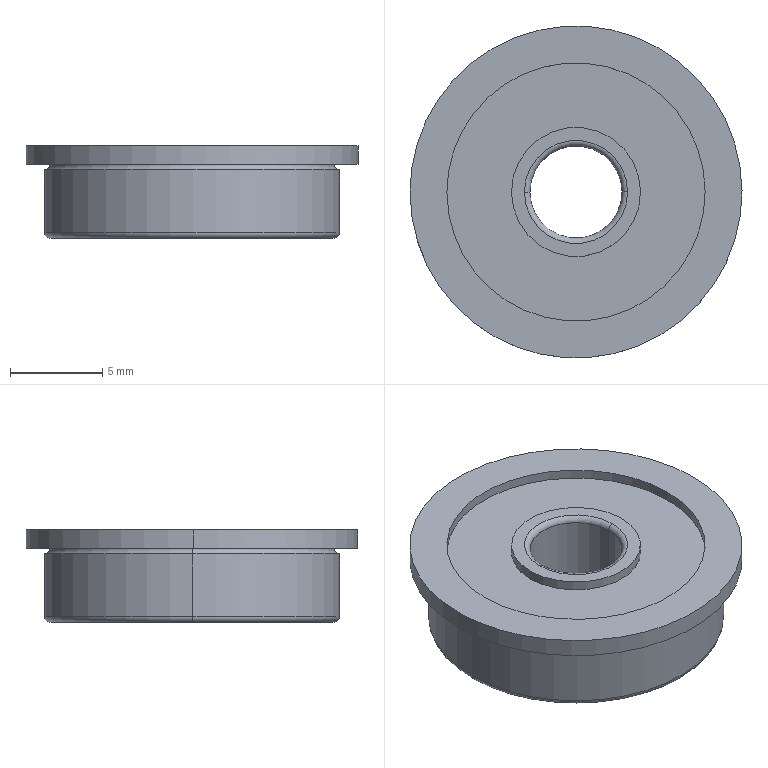Component | SolidWorks | SL010-LeftStreamline-1-1_SL010-PulleyAssembly-1-2_SL010-FL625ZZ-1-2 | 1 solid | 31 faces | box 18 x 18 x 5 mm | volume 827 mm3 | cylinder 14 | torus 10 | plane 7 | commonest cylinder face diameters 7 x4 14 x4 16 x2 18 x2 5 x2
STEP:
#1=COLOUR_RGB('',0.7922,0.8196,0.9333);
#2=FILL_AREA_STYLE_COLOUR('',#1);
#3=FILL_AREA_STYLE('',(#2));
#4=SURFACE_STYLE_FILL_AREA(#3);
#5=SURFACE_SIDE_STYLE('',(#4));
#6=SURFACE_STYLE_USAGE(.BOTH.,#5);
#7=PRESENTATION_STYLE_ASSIGNMENT((#6));
#8=CARTESIAN_POINT('',(-29.594,-5.329,-24.923));
#9=VERTEX_POINT('',#8);
#10=CARTESIAN_POINT('',(-29.618,-5.329,-24.923));
#11=VERTEX_POINT('',#10);
#12=CARTESIAN_POINT('',(-29.594,-5.329,-24.923));
#13=CARTESIAN_POINT('',(-29.594,-5.329,-24.92));
#14=CARTESIAN_POINT('',(-29.596,-5.329,-24.916));
#15=CARTESIAN_POINT('',(-29.6,-5.329,-24.912));
#16=CARTESIAN_POINT('',(-29.603,-5.329,-24.911));
#17=CARTESIAN_POINT('',(-29.609,-5.329,-24.911));
#18=CARTESIAN_POINT('',(-29.612,-5.329,-24.912));
#19=CARTESIAN_POINT('',(-29.617,-5.329,-24.916));
#20=CARTESIAN_POINT('',(-29.618,-5.329,-24.92));
#21=CARTESIAN_POINT('',(-29.618,-5.329,-24.923));
#22=B_SPLINE_CURVE_WITH_KNOTS('',3,(#12,#13,#14,#15,#16,#17,#18,#19,#20,#21),.UNSPECIFIED.,.F.,.F.,(4,2,2,2,4),(0.,0.7854,1.571,2.356,3.142),.UNSPECIFIED.);
#23=EDGE_CURVE('',#9,#11,#22,.T.);
#24=ORIENTED_EDGE('',*,*,#23,.T.);
#25=CARTESIAN_POINT('',(-30.224,-5.333,-24.923));
#26=VERTEX_POINT('',#25);
#27=CARTESIAN_POINT('',(-29.921,-5.331,-24.923));
#28=DIRECTION('',(0.,0.,1.));
#29=DIRECTION('',(0.,-1.,0.));
#30=AXIS2_PLACEMENT_3D('',#27,#28,#29);
#31=CIRCLE('',#30,0.3031);
#32=EDGE_CURVE('',#11,#26,#31,.T.);
#33=ORIENTED_EDGE('',*,*,#32,.T.);
#34=CARTESIAN_POINT('',(-30.248,-5.333,-24.923));
#35=VERTEX_POINT('',#34);
#36=CARTESIAN_POINT('',(-30.248,-5.333,-24.923));
#37=CARTESIAN_POINT('',(-30.248,-5.333,-24.92));
#38=CARTESIAN_POINT('',(-30.247,-5.333,-24.916));
#39=CARTESIAN_POINT('',(-30.242,-5.333,-24.912));
#40=CARTESIAN_POINT('',(-30.239,-5.333,-24.911));
#41=CARTESIAN_POINT('',(-30.233,-5.333,-24.911));
#42=CARTESIAN_POINT('',(-30.23,-5.333,-24.912));
#43=CARTESIAN_POINT('',(-30.226,-5.333,-24.916));
#44=CARTESIAN_POINT('',(-30.224,-5.333,-24.92));
#45=CARTESIAN_POINT('',(-30.224,-5.333,-24.923));
#46=B_SPLINE_CURVE_WITH_KNOTS('',3,(#36,#37,#38,#39,#40,#41,#42,#43,#44,#45),.UNSPECIFIED.,.F.,.F.,(4,2,2,2,4),(0.,0.7854,1.571,2.356,3.142),.UNSPECIFIED.);
#47=EDGE_CURVE('',#35,#26,#46,.T.);
#48=ORIENTED_EDGE('',*,*,#47,.F.);
#49=CARTESIAN_POINT('',(-29.921,-5.331,-24.923));
#50=DIRECTION('',(0.,0.,1.));
#51=DIRECTION('',(1.,0.006701,0.));
#52=AXIS2_PLACEMENT_3D('',#49,#50,#51);
#53=CIRCLE('',#52,0.3268);
#54=EDGE_CURVE('',#9,#35,#53,.T.);
#55=ORIENTED_EDGE('',*,*,#54,.F.);
#56=EDGE_LOOP('',(#24,#33,#48,#55));
#57=FACE_OUTER_BOUND('',#56,.T.);
#58=CARTESIAN_POINT('',(-29.921,-5.331,-24.923));
#59=DIRECTION('',(0.,0.,1.));
#60=DIRECTION('',(0.006701,-1.,0.));
#61=AXIS2_PLACEMENT_3D('',#58,#59,#60);
#62=TOROIDAL_SURFACE('',#61,0.315,0.01181);
#63=ADVANCED_FACE('',(#57),#62,.F.);
#64=ORIENTED_EDGE('',*,*,#47,.T.);
#65=CARTESIAN_POINT('',(-29.921,-5.331,-24.923));
#66=DIRECTION('',(0.,0.,1.));
#67=DIRECTION('',(0.,-1.,0.));
#68=AXIS2_PLACEMENT_3D('',#65,#66,#67);
#69=CIRCLE('',#68,0.3031);
#70=EDGE_CURVE('',#26,#11,#69,.T.);
#71=ORIENTED_EDGE('',*,*,#70,.T.);
#72=ORIENTED_EDGE('',*,*,#23,.F.);
#73=CARTESIAN_POINT('',(-29.921,-5.331,-24.923));
#74=DIRECTION('',(0.,0.,1.));
#75=DIRECTION('',(1.,0.006701,0.));
#76=AXIS2_PLACEMENT_3D('',#73,#74,#75);
#77=CIRCLE('',#76,0.3268);
#78=EDGE_CURVE('',#35,#9,#77,.T.);
#79=ORIENTED_EDGE('',*,*,#78,.F.);
#80=EDGE_LOOP('',(#64,#71,#72,#79));
#81=FACE_OUTER_BOUND('',#80,.T.);
#82=CARTESIAN_POINT('',(-29.921,-5.331,-24.923));
#83=DIRECTION('',(0.,0.,1.));
#84=DIRECTION('',(-0.006701,1.,-0.));
#85=AXIS2_PLACEMENT_3D('',#82,#83,#84);
#86=TOROIDAL_SURFACE('',#85,0.315,0.01181);
#87=ADVANCED_FACE('',(#81),#86,.F.);
#88=CARTESIAN_POINT('',(-29.811,-5.33,-25.08));
#89=VERTEX_POINT('',#88);
#90=CARTESIAN_POINT('',(-30.031,-5.332,-25.08));
#91=VERTEX_POINT('',#90);
#92=CARTESIAN_POINT('',(-29.921,-5.331,-25.08));
#93=DIRECTION('',(0.,0.,1.));
#94=DIRECTION('',(1.,0.006701,0.));
#95=AXIS2_PLACEMENT_3D('',#92,#93,#94);
#96=CIRCLE('',#95,0.1102);
#97=EDGE_CURVE('',#89,#91,#96,.T.);
#98=ORIENTED_EDGE('',*,*,#97,.T.);
#99=CARTESIAN_POINT('',(-29.921,-5.331,-25.08));
#100=DIRECTION('',(0.,0.,1.));
#101=DIRECTION('',(1.,0.006701,0.));
#102=AXIS2_PLACEMENT_3D('',#99,#100,#101);
#103=CIRCLE('',#102,0.1102);
#104=EDGE_CURVE('',#91,#89,#103,.T.);
#105=ORIENTED_EDGE('',*,*,#104,.T.);
#106=EDGE_LOOP('',(#98,#105));
#107=FACE_BOUND('',#106,.T.);
#108=CARTESIAN_POINT('',(-29.783,-5.33,-25.08));
#109=VERTEX_POINT('',#108);
#110=CARTESIAN_POINT('',(-30.059,-5.332,-25.08));
#111=VERTEX_POINT('',#110);
#112=CARTESIAN_POINT('',(-29.921,-5.331,-25.08));
#113=DIRECTION('',(0.,0.,1.));
#114=DIRECTION('',(1.,0.006701,0.));
#115=AXIS2_PLACEMENT_3D('',#112,#113,#114);
#116=CIRCLE('',#115,0.1378);
#117=EDGE_CURVE('',#109,#111,#116,.T.);
#118=ORIENTED_EDGE('',*,*,#117,.F.);
#119=CARTESIAN_POINT('',(-29.921,-5.331,-25.08));
#120=DIRECTION('',(0.,0.,1.));
#121=DIRECTION('',(1.,0.006701,0.));
#122=AXIS2_PLACEMENT_3D('',#119,#120,#121);
#123=CIRCLE('',#122,0.1378);
#124=EDGE_CURVE('',#111,#109,#123,.T.);
#125=ORIENTED_EDGE('',*,*,#124,.F.);
#126=EDGE_LOOP('',(#118,#125));
#127=FACE_OUTER_BOUND('',#126,.T.);
#128=CARTESIAN_POINT('',(-29.922,-5.193,-25.08));
#129=DIRECTION('',(-0.,-0.,-1.));
#130=DIRECTION('',(-1.,-0.006701,0.));
#131=AXIS2_PLACEMENT_3D('',#128,#129,#130);
#132=PLANE('',#131);
#133=ADVANCED_FACE('',(#107,#127),#132,.T.);
#134=ORIENTED_EDGE('',*,*,#124,.T.);
#135=CARTESIAN_POINT('',(-29.783,-5.33,-25.06));
#136=VERTEX_POINT('',#135);
#137=CARTESIAN_POINT('',(-29.783,-5.33,-25.06));
#138=CARTESIAN_POINT('',(-29.783,-5.33,-25.066));
#139=CARTESIAN_POINT('',(-29.783,-5.33,-25.073));
#140=CARTESIAN_POINT('',(-29.783,-5.33,-25.08));
#141=B_SPLINE_CURVE_WITH_KNOTS('',3,(#137,#138,#139,#140),.UNSPECIFIED.,.F.,.F.,(4,4),(15.476,16.),.UNSPECIFIED.);
#142=EDGE_CURVE('',#136,#109,#141,.T.);
#143=ORIENTED_EDGE('',*,*,#142,.F.);
#144=CARTESIAN_POINT('',(-30.059,-5.332,-25.06));
#145=VERTEX_POINT('',#144);
#146=CARTESIAN_POINT('',(-29.921,-5.331,-25.06));
#147=DIRECTION('',(0.,0.,1.));
#148=DIRECTION('',(1.,0.006701,0.));
#149=AXIS2_PLACEMENT_3D('',#146,#147,#148);
#150=CIRCLE('',#149,0.1378);
#151=EDGE_CURVE('',#145,#136,#150,.T.);
#152=ORIENTED_EDGE('',*,*,#151,.F.);
#153=CARTESIAN_POINT('',(-30.059,-5.332,-25.06));
#154=CARTESIAN_POINT('',(-30.059,-5.332,-25.066));
#155=CARTESIAN_POINT('',(-30.059,-5.332,-25.073));
#156=CARTESIAN_POINT('',(-30.059,-5.332,-25.08));
#157=B_SPLINE_CURVE_WITH_KNOTS('',3,(#153,#154,#155,#156),.UNSPECIFIED.,.F.,.F.,(4,4),(15.476,16.),.UNSPECIFIED.);
#158=EDGE_CURVE('',#145,#111,#157,.T.);
#159=ORIENTED_EDGE('',*,*,#158,.T.);
#160=EDGE_LOOP('',(#134,#143,#152,#159));
#161=FACE_OUTER_BOUND('',#160,.T.);
#162=CARTESIAN_POINT('',(-29.921,-5.331,-24.45));
#163=DIRECTION('',(-0.,-0.,-1.));
#164=DIRECTION('',(-0.006701,1.,0.));
#165=AXIS2_PLACEMENT_3D('',#162,#163,#164);
#166=CYLINDRICAL_SURFACE('',#165,0.1378);
#167=ADVANCED_FACE('',(#161),#166,.T.);
#168=CARTESIAN_POINT('',(-29.921,-5.331,-25.06));
#169=DIRECTION('',(0.,0.,1.));
#170=DIRECTION('',(1.,0.006701,0.));
#171=AXIS2_PLACEMENT_3D('',#168,#169,#170);
#172=CIRCLE('',#171,0.1378);
#173=EDGE_CURVE('',#136,#145,#172,.T.);
#174=ORIENTED_EDGE('',*,*,#173,.F.);
#175=ORIENTED_EDGE('',*,*,#142,.T.);
#176=ORIENTED_EDGE('',*,*,#117,.T.);
#177=ORIENTED_EDGE('',*,*,#158,.F.);
#178=EDGE_LOOP('',(#174,#175,#176,#177));
#179=FACE_OUTER_BOUND('',#178,.T.);
#180=CARTESIAN_POINT('',(-29.921,-5.331,-24.45));
#181=DIRECTION('',(-0.,-0.,-1.));
#182=DIRECTION('',(0.006701,-1.,0.));
#183=AXIS2_PLACEMENT_3D('',#180,#181,#182);
#184=CYLINDRICAL_SURFACE('',#183,0.1378);
#185=ADVANCED_FACE('',(#179),#184,.T.);
#186=ORIENTED_EDGE('',*,*,#173,.T.);
#187=ORIENTED_EDGE('',*,*,#151,.T.);
#188=EDGE_LOOP('',(#186,#187));
#189=FACE_BOUND('',#188,.T.);
#190=CARTESIAN_POINT('',(-29.646,-5.329,-25.06));
#191=VERTEX_POINT('',#190);
#192=CARTESIAN_POINT('',(-30.197,-5.333,-25.06));
#193=VERTEX_POINT('',#192);
#194=CARTESIAN_POINT('',(-29.921,-5.331,-25.06));
#195=DIRECTION('',(0.,0.,1.));
#196=DIRECTION('',(1.,0.006701,0.));
#197=AXIS2_PLACEMENT_3D('',#194,#195,#196);
#198=CIRCLE('',#197,0.2756);
#199=EDGE_CURVE('',#191,#193,#198,.T.);
#200=ORIENTED_EDGE('',*,*,#199,.F.);
#201=CARTESIAN_POINT('',(-29.921,-5.331,-25.06));
#202=DIRECTION('',(0.,0.,1.));
#203=DIRECTION('',(1.,0.006701,0.));
#204=AXIS2_PLACEMENT_3D('',#201,#202,#203);
#205=CIRCLE('',#204,0.2756);
#206=EDGE_CURVE('',#193,#191,#205,.T.);
#207=ORIENTED_EDGE('',*,*,#206,.F.);
#208=EDGE_LOOP('',(#200,#207));
#209=FACE_OUTER_BOUND('',#208,.T.);
#210=CARTESIAN_POINT('',(-29.923,-5.055,-25.06));
#211=DIRECTION('',(-0.,-0.,-1.));
#212=DIRECTION('',(-1.,-0.006701,0.));
#213=AXIS2_PLACEMENT_3D('',#210,#211,#212);
#214=PLANE('',#213);
#215=ADVANCED_FACE('',(#189,#209),#214,.T.);
#216=CARTESIAN_POINT('',(-30.197,-5.333,-25.08));
#217=VERTEX_POINT('',#216);
#218=CARTESIAN_POINT('',(-29.646,-5.329,-25.08));
#219=VERTEX_POINT('',#218);
#220=CARTESIAN_POINT('',(-29.921,-5.331,-25.08));
#221=DIRECTION('',(0.,0.,1.));
#222=DIRECTION('',(1.,0.006701,0.));
#223=AXIS2_PLACEMENT_3D('',#220,#221,#222);
#224=CIRCLE('',#223,0.2756);
#225=EDGE_CURVE('',#217,#219,#224,.T.);
#226=ORIENTED_EDGE('',*,*,#225,.F.);
#227=CARTESIAN_POINT('',(-30.197,-5.333,-25.06));
#228=CARTESIAN_POINT('',(-30.197,-5.333,-25.066));
#229=CARTESIAN_POINT('',(-30.197,-5.333,-25.073));
#230=CARTESIAN_POINT('',(-30.197,-5.333,-25.08));
#231=B_SPLINE_CURVE_WITH_KNOTS('',3,(#227,#228,#229,#230),.UNSPECIFIED.,.F.,.F.,(4,4),(15.476,16.),.UNSPECIFIED.);
#232=EDGE_CURVE('',#193,#217,#231,.T.);
#233=ORIENTED_EDGE('',*,*,#232,.F.);
#234=ORIENTED_EDGE('',*,*,#206,.T.);
#235=CARTESIAN_POINT('',(-29.646,-5.329,-25.06));
#236=CARTESIAN_POINT('',(-29.646,-5.329,-25.066));
#237=CARTESIAN_POINT('',(-29.646,-5.329,-25.073));
#238=CARTESIAN_POINT('',(-29.646,-5.329,-25.08));
#239=B_SPLINE_CURVE_WITH_KNOTS('',3,(#235,#236,#237,#238),.UNSPECIFIED.,.F.,.F.,(4,4),(15.476,16.),.UNSPECIFIED.);
#240=EDGE_CURVE('',#191,#219,#239,.T.);
#241=ORIENTED_EDGE('',*,*,#240,.T.);
#242=EDGE_LOOP('',(#226,#233,#234,#241));
#243=FACE_OUTER_BOUND('',#242,.T.);
#244=CARTESIAN_POINT('',(-29.921,-5.331,-24.45));
#245=DIRECTION('',(-0.,-0.,-1.));
#246=DIRECTION('',(-0.006701,1.,0.));
#247=AXIS2_PLACEMENT_3D('',#244,#245,#246);
#248=CYLINDRICAL_SURFACE('',#247,0.2756);
#249=ADVANCED_FACE('',(#243),#248,.F.);
#250=ORIENTED_EDGE('',*,*,#199,.T.);
#251=ORIENTED_EDGE('',*,*,#232,.T.);
#252=CARTESIAN_POINT('',(-29.921,-5.331,-25.08));
#253=DIRECTION('',(0.,0.,1.));
#254=DIRECTION('',(1.,0.006701,0.));
#255=AXIS2_PLACEMENT_3D('',#252,#253,#254);
#256=CIRCLE('',#255,0.2756);
#257=EDGE_CURVE('',#219,#217,#256,.T.);
#258=ORIENTED_EDGE('',*,*,#257,.F.);
#259=ORIENTED_EDGE('',*,*,#240,.F.);
#260=EDGE_LOOP('',(#250,#251,#258,#259));
#261=FACE_OUTER_BOUND('',#260,.T.);
#262=CARTESIAN_POINT('',(-29.921,-5.331,-24.45));
#263=DIRECTION('',(-0.,-0.,-1.));
#264=DIRECTION('',(0.006701,-1.,0.));
#265=AXIS2_PLACEMENT_3D('',#262,#263,#264);
#266=CYLINDRICAL_SURFACE('',#265,0.2756);
#267=ADVANCED_FACE('',(#261),#266,.F.);
#268=ORIENTED_EDGE('',*,*,#257,.T.);
#269=ORIENTED_EDGE('',*,*,#225,.T.);
#270=EDGE_LOOP('',(#268,#269));
#271=FACE_BOUND('',#270,.T.);
#272=CARTESIAN_POINT('',(-29.618,-5.329,-25.08));
#273=VERTEX_POINT('',#272);
#274=CARTESIAN_POINT('',(-30.224,-5.333,-25.08));
#275=VERTEX_POINT('',#274);
#276=CARTESIAN_POINT('',(-29.921,-5.331,-25.08));
#277=DIRECTION('',(0.,0.,1.));
#278=DIRECTION('',(1.,0.006701,0.));
#279=AXIS2_PLACEMENT_3D('',#276,#277,#278);
#280=CIRCLE('',#279,0.3031);
#281=EDGE_CURVE('',#273,#275,#280,.T.);
#282=ORIENTED_EDGE('',*,*,#281,.F.);
#283=CARTESIAN_POINT('',(-29.921,-5.331,-25.08));
#284=DIRECTION('',(0.,0.,1.));
#285=DIRECTION('',(1.,0.006701,0.));
#286=AXIS2_PLACEMENT_3D('',#283,#284,#285);
#287=CIRCLE('',#286,0.3031);
#288=EDGE_CURVE('',#275,#273,#287,.T.);
#289=ORIENTED_EDGE('',*,*,#288,.F.);
#290=EDGE_LOOP('',(#282,#289));
#291=FACE_OUTER_BOUND('',#290,.T.);
#292=CARTESIAN_POINT('',(-29.923,-5.028,-25.08));
#293=DIRECTION('',(-0.,-0.,-1.));
#294=DIRECTION('',(-1.,-0.006701,0.));
#295=AXIS2_PLACEMENT_3D('',#292,#293,#294);
#296=PLANE('',#295);
#297=ADVANCED_FACE('',(#271,#291),#296,.T.);
#298=ORIENTED_EDGE('',*,*,#288,.T.);
#299=CARTESIAN_POINT('',(-29.606,-5.329,-25.068));
#300=VERTEX_POINT('',#299);
#301=CARTESIAN_POINT('',(-29.618,-5.329,-25.08));
#302=CARTESIAN_POINT('',(-29.615,-5.329,-25.08));
#303=CARTESIAN_POINT('',(-29.612,-5.329,-25.079));
#304=CARTESIAN_POINT('',(-29.608,-5.329,-25.074));
#305=CARTESIAN_POINT('',(-29.606,-5.329,-25.071));
#306=CARTESIAN_POINT('',(-29.606,-5.329,-25.068));
#307=B_SPLINE_CURVE_WITH_KNOTS('',3,(#301,#302,#303,#304,#305,#306),.UNSPECIFIED.,.F.,.F.,(4,2,4),(0.,0.7854,1.571),.UNSPECIFIED.);
#308=EDGE_CURVE('',#273,#300,#307,.T.);
#309=ORIENTED_EDGE('',*,*,#308,.T.);
#310=CARTESIAN_POINT('',(-30.236,-5.333,-25.068));
#311=VERTEX_POINT('',#310);
#312=CARTESIAN_POINT('',(-29.921,-5.331,-25.068));
#313=DIRECTION('',(0.,0.,1.));
#314=DIRECTION('',(1.,0.006701,0.));
#315=AXIS2_PLACEMENT_3D('',#312,#313,#314);
#316=CIRCLE('',#315,0.315);
#317=EDGE_CURVE('',#311,#300,#316,.T.);
#318=ORIENTED_EDGE('',*,*,#317,.F.);
#319=CARTESIAN_POINT('',(-30.224,-5.333,-25.08));
#320=CARTESIAN_POINT('',(-30.227,-5.333,-25.08));
#321=CARTESIAN_POINT('',(-30.231,-5.333,-25.079));
#322=CARTESIAN_POINT('',(-30.235,-5.333,-25.074));
#323=CARTESIAN_POINT('',(-30.236,-5.333,-25.071));
#324=CARTESIAN_POINT('',(-30.236,-5.333,-25.068));
#325=B_SPLINE_CURVE_WITH_KNOTS('',3,(#319,#320,#321,#322,#323,#324),.UNSPECIFIED.,.F.,.F.,(4,2,4),(0.,0.7854,1.571),.UNSPECIFIED.);
#326=EDGE_CURVE('',#275,#311,#325,.T.);
#327=ORIENTED_EDGE('',*,*,#326,.F.);
#328=EDGE_LOOP('',(#298,#309,#318,#327));
#329=FACE_OUTER_BOUND('',#328,.T.);
#330=CARTESIAN_POINT('',(-29.921,-5.331,-25.068));
#331=DIRECTION('',(0.,0.,1.));
#332=DIRECTION('',(-0.006701,1.,-0.));
#333=AXIS2_PLACEMENT_3D('',#330,#331,#332);
#334=TOROIDAL_SURFACE('',#333,0.3031,0.01181);
#335=ADVANCED_FACE('',(#329),#334,.T.);
#336=CARTESIAN_POINT('',(-29.921,-5.331,-25.068));
#337=DIRECTION('',(0.,0.,1.));
#338=DIRECTION('',(1.,0.006701,0.));
#339=AXIS2_PLACEMENT_3D('',#336,#337,#338);
#340=CIRCLE('',#339,0.315);
#341=EDGE_CURVE('',#300,#311,#340,.T.);
#342=ORIENTED_EDGE('',*,*,#341,.F.);
#343=ORIENTED_EDGE('',*,*,#308,.F.);
#344=ORIENTED_EDGE('',*,*,#281,.T.);
#345=ORIENTED_EDGE('',*,*,#326,.T.);
#346=EDGE_LOOP('',(#342,#343,#344,#345));
#347=FACE_OUTER_BOUND('',#346,.T.);
#348=CARTESIAN_POINT('',(-29.921,-5.331,-25.068));
#349=DIRECTION('',(0.,0.,1.));
#350=DIRECTION('',(0.006701,-1.,0.));
#351=AXIS2_PLACEMENT_3D('',#348,#349,#350);
#352=TOROIDAL_SURFACE('',#351,0.3031,0.01181);
#353=ADVANCED_FACE('',(#347),#352,.T.);
#354=CARTESIAN_POINT('',(-29.606,-5.329,-24.934));
#355=VERTEX_POINT('',#354);
#356=CARTESIAN_POINT('',(-30.236,-5.333,-24.934));
#357=VERTEX_POINT('',#356);
#358=CARTESIAN_POINT('',(-29.921,-5.331,-24.934));
#359=DIRECTION('',(0.,0.,1.));
#360=DIRECTION('',(1.,0.006701,0.));
#361=AXIS2_PLACEMENT_3D('',#358,#359,#360);
#362=CIRCLE('',#361,0.315);
#363=EDGE_CURVE('',#355,#357,#362,.T.);
#364=ORIENTED_EDGE('',*,*,#363,.F.);
#365=CARTESIAN_POINT('',(-29.606,-5.329,-24.934));
#366=CARTESIAN_POINT('',(-29.606,-5.329,-24.979));
#367=CARTESIAN_POINT('',(-29.606,-5.329,-25.024));
#368=CARTESIAN_POINT('',(-29.606,-5.329,-25.068));
#369=B_SPLINE_CURVE_WITH_KNOTS('',3,(#365,#366,#367,#368),.UNSPECIFIED.,.F.,.F.,(4,4),(12.3,15.7),.UNSPECIFIED.);
#370=EDGE_CURVE('',#355,#300,#369,.T.);
#371=ORIENTED_EDGE('',*,*,#370,.T.);
#372=ORIENTED_EDGE('',*,*,#341,.T.);
#373=CARTESIAN_POINT('',(-30.236,-5.333,-24.934));
#374=CARTESIAN_POINT('',(-30.236,-5.333,-24.979));
#375=CARTESIAN_POINT('',(-30.236,-5.333,-25.024));
#376=CARTESIAN_POINT('',(-30.236,-5.333,-25.068));
#377=B_SPLINE_CURVE_WITH_KNOTS('',3,(#373,#374,#375,#376),.UNSPECIFIED.,.F.,.F.,(4,4),(12.3,15.7),.UNSPECIFIED.);
#378=EDGE_CURVE('',#357,#311,#377,.T.);
#379=ORIENTED_EDGE('',*,*,#378,.F.);
#380=EDGE_LOOP('',(#364,#371,#372,#379));
#381=FACE_OUTER_BOUND('',#380,.T.);
#382=CARTESIAN_POINT('',(-29.921,-5.331,-24.45));
#383=DIRECTION('',(-0.,-0.,-1.));
#384=DIRECTION('',(0.006701,-1.,0.));
#385=AXIS2_PLACEMENT_3D('',#382,#383,#384);
#386=CYLINDRICAL_SURFACE('',#385,0.315);
#387=ADVANCED_FACE('',(#381),#386,.T.);
#388=ORIENTED_EDGE('',*,*,#317,.T.);
#389=ORIENTED_EDGE('',*,*,#370,.F.);
#390=CARTESIAN_POINT('',(-29.921,-5.331,-24.934));
#391=DIRECTION('',(0.,0.,1.));
#392=DIRECTION('',(1.,0.006701,0.));
#393=AXIS2_PLACEMENT_3D('',#390,#391,#392);
#394=CIRCLE('',#393,0.315);
#395=EDGE_CURVE('',#357,#355,#394,.T.);
#396=ORIENTED_EDGE('',*,*,#395,.F.);
#397=ORIENTED_EDGE('',*,*,#378,.T.);
#398=EDGE_LOOP('',(#388,#389,#396,#397));
#399=FACE_OUTER_BOUND('',#398,.T.);
#400=CARTESIAN_POINT('',(-29.921,-5.331,-24.45));
#401=DIRECTION('',(-0.,-0.,-1.));
#402=DIRECTION('',(-0.006701,1.,0.));
#403=AXIS2_PLACEMENT_3D('',#400,#401,#402);
#404=CYLINDRICAL_SURFACE('',#403,0.315);
#405=ADVANCED_FACE('',(#399),#404,.T.);
#406=ORIENTED_EDGE('',*,*,#70,.F.);
#407=CARTESIAN_POINT('',(-30.224,-5.333,-24.923));
#408=CARTESIAN_POINT('',(-30.224,-5.333,-24.926));
#409=CARTESIAN_POINT('',(-30.226,-5.333,-24.929));
#410=CARTESIAN_POINT('',(-30.23,-5.333,-24.933));
#411=CARTESIAN_POINT('',(-30.233,-5.333,-24.934));
#412=CARTESIAN_POINT('',(-30.236,-5.333,-24.934));
#413=B_SPLINE_CURVE_WITH_KNOTS('',3,(#407,#408,#409,#410,#411,#412),.UNSPECIFIED.,.F.,.F.,(4,2,4),(3.142,3.927,4.712),.UNSPECIFIED.);
#414=EDGE_CURVE('',#26,#357,#413,.T.);
#415=ORIENTED_EDGE('',*,*,#414,.T.);
#416=ORIENTED_EDGE('',*,*,#395,.T.);
#417=CARTESIAN_POINT('',(-29.618,-5.329,-24.923));
#418=CARTESIAN_POINT('',(-29.618,-5.329,-24.926));
#419=CARTESIAN_POINT('',(-29.617,-5.329,-24.929));
#420=CARTESIAN_POINT('',(-29.612,-5.329,-24.933));
#421=CARTESIAN_POINT('',(-29.609,-5.329,-24.934));
#422=CARTESIAN_POINT('',(-29.606,-5.329,-24.934));
#423=B_SPLINE_CURVE_WITH_KNOTS('',3,(#417,#418,#419,#420,#421,#422),.UNSPECIFIED.,.F.,.F.,(4,2,4),(3.142,3.927,4.712),.UNSPECIFIED.);
#424=EDGE_CURVE('',#11,#355,#423,.T.);
#425=ORIENTED_EDGE('',*,*,#424,.F.);
#426=EDGE_LOOP('',(#406,#415,#416,#425));
#427=FACE_OUTER_BOUND('',#426,.T.);
#428=CARTESIAN_POINT('',(-29.921,-5.331,-24.923));
#429=DIRECTION('',(0.,0.,1.));
#430=DIRECTION('',(-0.006701,1.,-0.));
#431=AXIS2_PLACEMENT_3D('',#428,#429,#430);
#432=TOROIDAL_SURFACE('',#431,0.315,0.01181);
#433=ADVANCED_FACE('',(#427),#432,.F.);
#434=ORIENTED_EDGE('',*,*,#32,.F.);
#435=ORIENTED_EDGE('',*,*,#424,.T.);
#436=ORIENTED_EDGE('',*,*,#363,.T.);
#437=ORIENTED_EDGE('',*,*,#414,.F.);
#438=EDGE_LOOP('',(#434,#435,#436,#437));
#439=FACE_OUTER_BOUND('',#438,.T.);
#440=CARTESIAN_POINT('',(-29.921,-5.331,-24.923));
#441=DIRECTION('',(0.,0.,1.));
#442=DIRECTION('',(0.006701,-1.,0.));
#443=AXIS2_PLACEMENT_3D('',#440,#441,#442);
#444=TOROIDAL_SURFACE('',#443,0.315,0.01181);
#445=ADVANCED_FACE('',(#439),#444,.F.);
#446=ORIENTED_EDGE('',*,*,#54,.T.);
#447=ORIENTED_EDGE('',*,*,#78,.T.);
#448=EDGE_LOOP('',(#446,#447));
#449=FACE_BOUND('',#448,.T.);
#450=CARTESIAN_POINT('',(-29.567,-5.329,-24.923));
#451=VERTEX_POINT('',#450);
#452=CARTESIAN_POINT('',(-30.276,-5.333,-24.923));
#453=VERTEX_POINT('',#452);
#454=CARTESIAN_POINT('',(-29.921,-5.331,-24.923));
#455=DIRECTION('',(0.,0.,1.));
#456=DIRECTION('',(1.,0.006701,0.));
#457=AXIS2_PLACEMENT_3D('',#454,#455,#456);
#458=CIRCLE('',#457,0.3543);
#459=EDGE_CURVE('',#451,#453,#458,.T.);
#460=ORIENTED_EDGE('',*,*,#459,.F.);
#461=CARTESIAN_POINT('',(-29.921,-5.331,-24.923));
#462=DIRECTION('',(0.,0.,1.));
#463=DIRECTION('',(1.,0.006701,0.));
#464=AXIS2_PLACEMENT_3D('',#461,#462,#463);
#465=CIRCLE('',#464,0.3543);
#466=EDGE_CURVE('',#453,#451,#465,.T.);
#467=ORIENTED_EDGE('',*,*,#466,.F.);
#468=EDGE_LOOP('',(#460,#467));
#469=FACE_OUTER_BOUND('',#468,.T.);
#470=CARTESIAN_POINT('',(-29.924,-4.977,-24.923));
#471=DIRECTION('',(-0.,-0.,-1.));
#472=DIRECTION('',(-1.,-0.006701,0.));
#473=AXIS2_PLACEMENT_3D('',#470,#471,#472);
#474=PLANE('',#473);
#475=ADVANCED_FACE('',(#449,#469),#474,.T.);
#476=ORIENTED_EDGE('',*,*,#466,.T.);
#477=CARTESIAN_POINT('',(-29.567,-5.329,-24.883));
#478=VERTEX_POINT('',#477);
#479=CARTESIAN_POINT('',(-29.567,-5.329,-24.883));
#480=CARTESIAN_POINT('',(-29.567,-5.329,-24.896));
#481=CARTESIAN_POINT('',(-29.567,-5.329,-24.91));
#482=CARTESIAN_POINT('',(-29.567,-5.329,-24.923));
#483=B_SPLINE_CURVE_WITH_KNOTS('',3,(#479,#480,#481,#482),.UNSPECIFIED.,.F.,.F.,(4,4),(11.,12.),.UNSPECIFIED.);
#484=EDGE_CURVE('',#478,#451,#483,.T.);
#485=ORIENTED_EDGE('',*,*,#484,.F.);
#486=CARTESIAN_POINT('',(-30.276,-5.333,-24.883));
#487=VERTEX_POINT('',#486);
#488=CARTESIAN_POINT('',(-29.921,-5.331,-24.883));
#489=DIRECTION('',(0.,0.,1.));
#490=DIRECTION('',(1.,0.006701,0.));
#491=AXIS2_PLACEMENT_3D('',#488,#489,#490);
#492=CIRCLE('',#491,0.3543);
#493=EDGE_CURVE('',#487,#478,#492,.T.);
#494=ORIENTED_EDGE('',*,*,#493,.F.);
#495=CARTESIAN_POINT('',(-30.276,-5.333,-24.883));
#496=CARTESIAN_POINT('',(-30.276,-5.333,-24.896));
#497=CARTESIAN_POINT('',(-30.276,-5.333,-24.91));
#498=CARTESIAN_POINT('',(-30.276,-5.333,-24.923));
#499=B_SPLINE_CURVE_WITH_KNOTS('',3,(#495,#496,#497,#498),.UNSPECIFIED.,.F.,.F.,(4,4),(11.,12.),.UNSPECIFIED.);
#500=EDGE_CURVE('',#487,#453,#499,.T.);
#501=ORIENTED_EDGE('',*,*,#500,.T.);
#502=EDGE_LOOP('',(#476,#485,#494,#501));
#503=FACE_OUTER_BOUND('',#502,.T.);
#504=CARTESIAN_POINT('',(-29.921,-5.331,-24.45));
#505=DIRECTION('',(-0.,-0.,-1.));
#506=DIRECTION('',(-0.006701,1.,0.));
#507=AXIS2_PLACEMENT_3D('',#504,#505,#506);
#508=CYLINDRICAL_SURFACE('',#507,0.3543);
#509=ADVANCED_FACE('',(#503),#508,.T.);
#510=CARTESIAN_POINT('',(-29.921,-5.331,-24.883));
#511=DIRECTION('',(0.,0.,1.));
#512=DIRECTION('',(1.,0.006701,0.));
#513=AXIS2_PLACEMENT_3D('',#510,#511,#512);
#514=CIRCLE('',#513,0.3543);
#515=EDGE_CURVE('',#478,#487,#514,.T.);
#516=ORIENTED_EDGE('',*,*,#515,.F.);
#517=ORIENTED_EDGE('',*,*,#484,.T.);
#518=ORIENTED_EDGE('',*,*,#459,.T.);
#519=ORIENTED_EDGE('',*,*,#500,.F.);
#520=EDGE_LOOP('',(#516,#517,#518,#519));
#521=FACE_OUTER_BOUND('',#520,.T.);
#522=CARTESIAN_POINT('',(-29.921,-5.331,-24.45));
#523=DIRECTION('',(-0.,-0.,-1.));
#524=DIRECTION('',(0.006701,-1.,0.));
#525=AXIS2_PLACEMENT_3D('',#522,#523,#524);
#526=CYLINDRICAL_SURFACE('',#525,0.3543);
#527=ADVANCED_FACE('',(#521),#526,.T.);
#528=ORIENTED_EDGE('',*,*,#515,.T.);
#529=ORIENTED_EDGE('',*,*,#493,.T.);
#530=EDGE_LOOP('',(#528,#529));
#531=FACE_OUTER_BOUND('',#530,.T.);
#532=CARTESIAN_POINT('',(-29.646,-5.329,-24.883));
#533=VERTEX_POINT('',#532);
#534=CARTESIAN_POINT('',(-30.197,-5.333,-24.883));
#535=VERTEX_POINT('',#534);
#536=CARTESIAN_POINT('',(-29.921,-5.331,-24.883));
#537=DIRECTION('',(0.,0.,1.));
#538=DIRECTION('',(1.,0.006701,0.));
#539=AXIS2_PLACEMENT_3D('',#536,#537,#538);
#540=CIRCLE('',#539,0.2756);
#541=EDGE_CURVE('',#533,#535,#540,.T.);
#542=ORIENTED_EDGE('',*,*,#541,.F.);
#543=CARTESIAN_POINT('',(-29.921,-5.331,-24.883));
#544=DIRECTION('',(0.,0.,1.));
#545=DIRECTION('',(1.,0.006701,0.));
#546=AXIS2_PLACEMENT_3D('',#543,#544,#545);
#547=CIRCLE('',#546,0.2756);
#548=EDGE_CURVE('',#535,#533,#547,.T.);
#549=ORIENTED_EDGE('',*,*,#548,.F.);
#550=EDGE_LOOP('',(#542,#549));
#551=FACE_BOUND('',#550,.T.);
#552=CARTESIAN_POINT('',(-29.923,-5.055,-24.883));
#553=DIRECTION('',(0.,0.,1.));
#554=DIRECTION('',(1.,0.006701,-0.));
#555=AXIS2_PLACEMENT_3D('',#552,#553,#554);
#556=PLANE('',#555);
#557=ADVANCED_FACE('',(#531,#551),#556,.T.);
#558=CARTESIAN_POINT('',(-30.197,-5.333,-24.904));
#559=VERTEX_POINT('',#558);
#560=CARTESIAN_POINT('',(-29.646,-5.329,-24.904));
#561=VERTEX_POINT('',#560);
#562=CARTESIAN_POINT('',(-29.921,-5.331,-24.904));
#563=DIRECTION('',(0.,0.,1.));
#564=DIRECTION('',(1.,0.006701,0.));
#565=AXIS2_PLACEMENT_3D('',#562,#563,#564);
#566=CIRCLE('',#565,0.2756);
#567=EDGE_CURVE('',#559,#561,#566,.T.);
#568=ORIENTED_EDGE('',*,*,#567,.F.);
#569=CARTESIAN_POINT('',(-30.197,-5.333,-24.883));
#570=CARTESIAN_POINT('',(-30.197,-5.333,-24.89));
#571=CARTESIAN_POINT('',(-30.197,-5.333,-24.897));
#572=CARTESIAN_POINT('',(-30.197,-5.333,-24.904));
#573=B_SPLINE_CURVE_WITH_KNOTS('',3,(#569,#570,#571,#572),.UNSPECIFIED.,.F.,.F.,(4,4),(11.,11.524),.UNSPECIFIED.);
#574=EDGE_CURVE('',#535,#559,#573,.T.);
#575=ORIENTED_EDGE('',*,*,#574,.F.);
#576=ORIENTED_EDGE('',*,*,#548,.T.);
#577=CARTESIAN_POINT('',(-29.646,-5.329,-24.883));
#578=CARTESIAN_POINT('',(-29.646,-5.329,-24.89));
#579=CARTESIAN_POINT('',(-29.646,-5.329,-24.897));
#580=CARTESIAN_POINT('',(-29.646,-5.329,-24.904));
#581=B_SPLINE_CURVE_WITH_KNOTS('',3,(#577,#578,#579,#580),.UNSPECIFIED.,.F.,.F.,(4,4),(11.,11.524),.UNSPECIFIED.);
#582=EDGE_CURVE('',#533,#561,#581,.T.);
#583=ORIENTED_EDGE('',*,*,#582,.T.);
#584=EDGE_LOOP('',(#568,#575,#576,#583));
#585=FACE_OUTER_BOUND('',#584,.T.);
#586=CARTESIAN_POINT('',(-29.921,-5.331,-24.45));
#587=DIRECTION('',(-0.,-0.,-1.));
#588=DIRECTION('',(-0.006701,1.,0.));
#589=AXIS2_PLACEMENT_3D('',#586,#587,#588);
#590=CYLINDRICAL_SURFACE('',#589,0.2756);
#591=ADVANCED_FACE('',(#585),#590,.F.);
#592=ORIENTED_EDGE('',*,*,#541,.T.);
#593=ORIENTED_EDGE('',*,*,#574,.T.);
#594=CARTESIAN_POINT('',(-29.921,-5.331,-24.904));
#595=DIRECTION('',(0.,0.,1.));
#596=DIRECTION('',(1.,0.006701,0.));
#597=AXIS2_PLACEMENT_3D('',#594,#595,#596);
#598=CIRCLE('',#597,0.2756);
#599=EDGE_CURVE('',#561,#559,#598,.T.);
#600=ORIENTED_EDGE('',*,*,#599,.F.);
#601=ORIENTED_EDGE('',*,*,#582,.F.);
#602=EDGE_LOOP('',(#592,#593,#600,#601));
#603=FACE_OUTER_BOUND('',#602,.T.);
#604=CARTESIAN_POINT('',(-29.921,-5.331,-24.45));
#605=DIRECTION('',(-0.,-0.,-1.));
#606=DIRECTION('',(0.006701,-1.,0.));
#607=AXIS2_PLACEMENT_3D('',#604,#605,#606);
#608=CYLINDRICAL_SURFACE('',#607,0.2756);
#609=ADVANCED_FACE('',(#603),#608,.F.);
#610=ORIENTED_EDGE('',*,*,#599,.T.);
#611=ORIENTED_EDGE('',*,*,#567,.T.);
#612=EDGE_LOOP('',(#610,#611));
#613=FACE_OUTER_BOUND('',#612,.T.);
#614=CARTESIAN_POINT('',(-29.783,-5.33,-24.904));
#615=VERTEX_POINT('',#614);
#616=CARTESIAN_POINT('',(-30.059,-5.332,-24.904));
#617=VERTEX_POINT('',#616);
#618=CARTESIAN_POINT('',(-29.921,-5.331,-24.904));
#619=DIRECTION('',(0.,0.,1.));
#620=DIRECTION('',(1.,0.006701,0.));
#621=AXIS2_PLACEMENT_3D('',#618,#619,#620);
#622=CIRCLE('',#621,0.1378);
#623=EDGE_CURVE('',#615,#617,#622,.T.);
#624=ORIENTED_EDGE('',*,*,#623,.F.);
#625=CARTESIAN_POINT('',(-29.921,-5.331,-24.904));
#626=DIRECTION('',(0.,0.,1.));
#627=DIRECTION('',(1.,0.006701,0.));
#628=AXIS2_PLACEMENT_3D('',#625,#626,#627);
#629=CIRCLE('',#628,0.1378);
#630=EDGE_CURVE('',#617,#615,#629,.T.);
#631=ORIENTED_EDGE('',*,*,#630,.F.);
#632=EDGE_LOOP('',(#624,#631));
#633=FACE_BOUND('',#632,.T.);
#634=CARTESIAN_POINT('',(-29.922,-5.193,-24.904));
#635=DIRECTION('',(0.,0.,1.));
#636=DIRECTION('',(1.,0.006701,-0.));
#637=AXIS2_PLACEMENT_3D('',#634,#635,#636);
#638=PLANE('',#637);
#639=ADVANCED_FACE('',(#613,#633),#638,.T.);
#640=ORIENTED_EDGE('',*,*,#630,.T.);
#641=CARTESIAN_POINT('',(-29.783,-5.33,-24.883));
#642=VERTEX_POINT('',#641);
#643=CARTESIAN_POINT('',(-29.783,-5.33,-24.883));
#644=CARTESIAN_POINT('',(-29.783,-5.33,-24.89));
#645=CARTESIAN_POINT('',(-29.783,-5.33,-24.897));
#646=CARTESIAN_POINT('',(-29.783,-5.33,-24.904));
#647=B_SPLINE_CURVE_WITH_KNOTS('',3,(#643,#644,#645,#646),.UNSPECIFIED.,.F.,.F.,(4,4),(11.,11.524),.UNSPECIFIED.);
#648=EDGE_CURVE('',#642,#615,#647,.T.);
#649=ORIENTED_EDGE('',*,*,#648,.F.);
#650=CARTESIAN_POINT('',(-30.059,-5.332,-24.883));
#651=VERTEX_POINT('',#650);
#652=CARTESIAN_POINT('',(-29.921,-5.331,-24.883));
#653=DIRECTION('',(0.,0.,1.));
#654=DIRECTION('',(1.,0.006701,0.));
#655=AXIS2_PLACEMENT_3D('',#652,#653,#654);
#656=CIRCLE('',#655,0.1378);
#657=EDGE_CURVE('',#651,#642,#656,.T.);
#658=ORIENTED_EDGE('',*,*,#657,.F.);
#659=CARTESIAN_POINT('',(-30.059,-5.332,-24.883));
#660=CARTESIAN_POINT('',(-30.059,-5.332,-24.89));
#661=CARTESIAN_POINT('',(-30.059,-5.332,-24.897));
#662=CARTESIAN_POINT('',(-30.059,-5.332,-24.904));
#663=B_SPLINE_CURVE_WITH_KNOTS('',3,(#659,#660,#661,#662),.UNSPECIFIED.,.F.,.F.,(4,4),(11.,11.524),.UNSPECIFIED.);
#664=EDGE_CURVE('',#651,#617,#663,.T.);
#665=ORIENTED_EDGE('',*,*,#664,.T.);
#666=EDGE_LOOP('',(#640,#649,#658,#665));
#667=FACE_OUTER_BOUND('',#666,.T.);
#668=CARTESIAN_POINT('',(-29.921,-5.331,-24.45));
#669=DIRECTION('',(-0.,-0.,-1.));
#670=DIRECTION('',(-0.006701,1.,0.));
#671=AXIS2_PLACEMENT_3D('',#668,#669,#670);
#672=CYLINDRICAL_SURFACE('',#671,0.1378);
#673=ADVANCED_FACE('',(#667),#672,.T.);
#674=CARTESIAN_POINT('',(-29.921,-5.331,-24.883));
#675=DIRECTION('',(0.,0.,1.));
#676=DIRECTION('',(1.,0.006701,0.));
#677=AXIS2_PLACEMENT_3D('',#674,#675,#676);
#678=CIRCLE('',#677,0.1378);
#679=EDGE_CURVE('',#642,#651,#678,.T.);
#680=ORIENTED_EDGE('',*,*,#679,.F.);
#681=ORIENTED_EDGE('',*,*,#648,.T.);
#682=ORIENTED_EDGE('',*,*,#623,.T.);
#683=ORIENTED_EDGE('',*,*,#664,.F.);
#684=EDGE_LOOP('',(#680,#681,#682,#683));
#685=FACE_OUTER_BOUND('',#684,.T.);
#686=CARTESIAN_POINT('',(-29.921,-5.331,-24.45));
#687=DIRECTION('',(-0.,-0.,-1.));
#688=DIRECTION('',(0.006701,-1.,0.));
#689=AXIS2_PLACEMENT_3D('',#686,#687,#688);
#690=CYLINDRICAL_SURFACE('',#689,0.1378);
#691=ADVANCED_FACE('',(#685),#690,.T.);
#692=ORIENTED_EDGE('',*,*,#679,.T.);
#693=ORIENTED_EDGE('',*,*,#657,.T.);
#694=EDGE_LOOP('',(#692,#693));
#695=FACE_OUTER_BOUND('',#694,.T.);
#696=CARTESIAN_POINT('',(-29.811,-5.33,-24.883));
#697=VERTEX_POINT('',#696);
#698=CARTESIAN_POINT('',(-30.031,-5.332,-24.883));
#699=VERTEX_POINT('',#698);
#700=CARTESIAN_POINT('',(-29.921,-5.331,-24.883));
#701=DIRECTION('',(0.,0.,1.));
#702=DIRECTION('',(1.,0.006701,0.));
#703=AXIS2_PLACEMENT_3D('',#700,#701,#702);
#704=CIRCLE('',#703,0.1102);
#705=EDGE_CURVE('',#697,#699,#704,.T.);
#706=ORIENTED_EDGE('',*,*,#705,.F.);
#707=CARTESIAN_POINT('',(-29.921,-5.331,-24.883));
#708=DIRECTION('',(0.,0.,1.));
#709=DIRECTION('',(1.,0.006701,0.));
#710=AXIS2_PLACEMENT_3D('',#707,#708,#709);
#711=CIRCLE('',#710,0.1102);
#712=EDGE_CURVE('',#699,#697,#711,.T.);
#713=ORIENTED_EDGE('',*,*,#712,.F.);
#714=EDGE_LOOP('',(#706,#713));
#715=FACE_BOUND('',#714,.T.);
#716=CARTESIAN_POINT('',(-29.922,-5.221,-24.883));
#717=DIRECTION('',(0.,0.,1.));
#718=DIRECTION('',(1.,0.006701,-0.));
#719=AXIS2_PLACEMENT_3D('',#716,#717,#718);
#720=PLANE('',#719);
#721=ADVANCED_FACE('',(#695,#715),#720,.T.);
#722=ORIENTED_EDGE('',*,*,#712,.T.);
#723=CARTESIAN_POINT('',(-29.823,-5.33,-24.895));
#724=VERTEX_POINT('',#723);
#725=CARTESIAN_POINT('',(-29.811,-5.33,-24.883));
#726=CARTESIAN_POINT('',(-29.814,-5.33,-24.883));
#727=CARTESIAN_POINT('',(-29.817,-5.33,-24.885));
#728=CARTESIAN_POINT('',(-29.822,-5.33,-24.889));
#729=CARTESIAN_POINT('',(-29.823,-5.33,-24.892));
#730=CARTESIAN_POINT('',(-29.823,-5.33,-24.895));
#731=B_SPLINE_CURVE_WITH_KNOTS('',3,(#725,#726,#727,#728,#729,#730),.UNSPECIFIED.,.F.,.F.,(4,2,4),(0.,0.7854,1.571),.UNSPECIFIED.);
#732=EDGE_CURVE('',#697,#724,#731,.T.);
#733=ORIENTED_EDGE('',*,*,#732,.T.);
#734=CARTESIAN_POINT('',(-30.02,-5.332,-24.895));
#735=VERTEX_POINT('',#734);
#736=CARTESIAN_POINT('',(-29.921,-5.331,-24.895));
#737=DIRECTION('',(0.,0.,1.));
#738=DIRECTION('',(1.,0.006701,0.));
#739=AXIS2_PLACEMENT_3D('',#736,#737,#738);
#740=CIRCLE('',#739,0.09843);
#741=EDGE_CURVE('',#735,#724,#740,.T.);
#742=ORIENTED_EDGE('',*,*,#741,.F.);
#743=CARTESIAN_POINT('',(-30.031,-5.332,-24.883));
#744=CARTESIAN_POINT('',(-30.028,-5.332,-24.883));
#745=CARTESIAN_POINT('',(-30.025,-5.332,-24.885));
#746=CARTESIAN_POINT('',(-30.021,-5.332,-24.889));
#747=CARTESIAN_POINT('',(-30.02,-5.332,-24.892));
#748=CARTESIAN_POINT('',(-30.02,-5.332,-24.895));
#749=B_SPLINE_CURVE_WITH_KNOTS('',3,(#743,#744,#745,#746,#747,#748),.UNSPECIFIED.,.F.,.F.,(4,2,4),(0.,0.7854,1.571),.UNSPECIFIED.);
#750=EDGE_CURVE('',#699,#735,#749,.T.);
#751=ORIENTED_EDGE('',*,*,#750,.F.);
#752=EDGE_LOOP('',(#722,#733,#742,#751));
#753=FACE_OUTER_BOUND('',#752,.T.);
#754=CARTESIAN_POINT('',(-29.921,-5.331,-24.895));
#755=DIRECTION('',(0.,0.,1.));
#756=DIRECTION('',(-0.006701,1.,-0.));
#757=AXIS2_PLACEMENT_3D('',#754,#755,#756);
#758=TOROIDAL_SURFACE('',#757,0.1102,0.01181);
#759=ADVANCED_FACE('',(#753),#758,.T.);
#760=CARTESIAN_POINT('',(-29.921,-5.331,-24.895));
#761=DIRECTION('',(0.,0.,1.));
#762=DIRECTION('',(1.,0.006701,0.));
#763=AXIS2_PLACEMENT_3D('',#760,#761,#762);
#764=CIRCLE('',#763,0.09843);
#765=EDGE_CURVE('',#724,#735,#764,.T.);
#766=ORIENTED_EDGE('',*,*,#765,.F.);
#767=ORIENTED_EDGE('',*,*,#732,.F.);
#768=ORIENTED_EDGE('',*,*,#705,.T.);
#769=ORIENTED_EDGE('',*,*,#750,.T.);
#770=EDGE_LOOP('',(#766,#767,#768,#769));
#771=FACE_OUTER_BOUND('',#770,.T.);
#772=CARTESIAN_POINT('',(-29.921,-5.331,-24.895));
#773=DIRECTION('',(0.,0.,1.));
#774=DIRECTION('',(0.006701,-1.,0.));
#775=AXIS2_PLACEMENT_3D('',#772,#773,#774);
#776=TOROIDAL_SURFACE('',#775,0.1102,0.01181);
#777=ADVANCED_FACE('',(#771),#776,.T.);
#778=ORIENTED_EDGE('',*,*,#765,.T.);
#779=CARTESIAN_POINT('',(-30.02,-5.332,-25.068));
#780=VERTEX_POINT('',#779);
#781=CARTESIAN_POINT('',(-30.02,-5.332,-24.895));
#782=CARTESIAN_POINT('',(-30.02,-5.332,-24.953));
#783=CARTESIAN_POINT('',(-30.02,-5.332,-25.011));
#784=CARTESIAN_POINT('',(-30.02,-5.332,-25.068));
#785=B_SPLINE_CURVE_WITH_KNOTS('',3,(#781,#782,#783,#784),.UNSPECIFIED.,.F.,.F.,(4,4),(11.3,15.7),.UNSPECIFIED.);
#786=EDGE_CURVE('',#735,#780,#785,.T.);
#787=ORIENTED_EDGE('',*,*,#786,.T.);
#788=CARTESIAN_POINT('',(-29.823,-5.33,-25.068));
#789=VERTEX_POINT('',#788);
#790=CARTESIAN_POINT('',(-29.921,-5.331,-25.068));
#791=DIRECTION('',(0.,0.,1.));
#792=DIRECTION('',(1.,0.006701,0.));
#793=AXIS2_PLACEMENT_3D('',#790,#791,#792);
#794=CIRCLE('',#793,0.09843);
#795=EDGE_CURVE('',#789,#780,#794,.T.);
#796=ORIENTED_EDGE('',*,*,#795,.F.);
#797=CARTESIAN_POINT('',(-29.823,-5.33,-24.895));
#798=CARTESIAN_POINT('',(-29.823,-5.33,-24.953));
#799=CARTESIAN_POINT('',(-29.823,-5.33,-25.011));
#800=CARTESIAN_POINT('',(-29.823,-5.33,-25.068));
#801=B_SPLINE_CURVE_WITH_KNOTS('',3,(#797,#798,#799,#800),.UNSPECIFIED.,.F.,.F.,(4,4),(11.3,15.7),.UNSPECIFIED.);
#802=EDGE_CURVE('',#724,#789,#801,.T.);
#803=ORIENTED_EDGE('',*,*,#802,.F.);
#804=EDGE_LOOP('',(#778,#787,#796,#803));
#805=FACE_OUTER_BOUND('',#804,.T.);
#806=CARTESIAN_POINT('',(-29.921,-5.331,-24.45));
#807=DIRECTION('',(-0.,-0.,-1.));
#808=DIRECTION('',(0.006701,-1.,0.));
#809=AXIS2_PLACEMENT_3D('',#806,#807,#808);
#810=CYLINDRICAL_SURFACE('',#809,0.09843);
#811=ADVANCED_FACE('',(#805),#810,.F.);
#812=CARTESIAN_POINT('',(-29.921,-5.331,-25.068));
#813=DIRECTION('',(0.,0.,1.));
#814=DIRECTION('',(1.,0.006701,0.));
#815=AXIS2_PLACEMENT_3D('',#812,#813,#814);
#816=CIRCLE('',#815,0.09843);
#817=EDGE_CURVE('',#780,#789,#816,.T.);
#818=ORIENTED_EDGE('',*,*,#817,.F.);
#819=ORIENTED_EDGE('',*,*,#786,.F.);
#820=ORIENTED_EDGE('',*,*,#741,.T.);
#821=ORIENTED_EDGE('',*,*,#802,.T.);
#822=EDGE_LOOP('',(#818,#819,#820,#821));
#823=FACE_OUTER_BOUND('',#822,.T.);
#824=CARTESIAN_POINT('',(-29.921,-5.331,-24.45));
#825=DIRECTION('',(-0.,-0.,-1.));
#826=DIRECTION('',(-0.006701,1.,0.));
#827=AXIS2_PLACEMENT_3D('',#824,#825,#826);
#828=CYLINDRICAL_SURFACE('',#827,0.09843);
#829=ADVANCED_FACE('',(#823),#828,.F.);
#830=ORIENTED_EDGE('',*,*,#817,.T.);
#831=CARTESIAN_POINT('',(-29.823,-5.33,-25.068));
#832=CARTESIAN_POINT('',(-29.823,-5.33,-25.071));
#833=CARTESIAN_POINT('',(-29.822,-5.33,-25.074));
#834=CARTESIAN_POINT('',(-29.817,-5.33,-25.079));
#835=CARTESIAN_POINT('',(-29.814,-5.33,-25.08));
#836=CARTESIAN_POINT('',(-29.811,-5.33,-25.08));
#837=B_SPLINE_CURVE_WITH_KNOTS('',3,(#831,#832,#833,#834,#835,#836),.UNSPECIFIED.,.F.,.F.,(4,2,4),(0.,0.7854,1.571),.UNSPECIFIED.);
#838=EDGE_CURVE('',#789,#89,#837,.T.);
#839=ORIENTED_EDGE('',*,*,#838,.T.);
#840=ORIENTED_EDGE('',*,*,#104,.F.);
#841=CARTESIAN_POINT('',(-30.02,-5.332,-25.068));
#842=CARTESIAN_POINT('',(-30.02,-5.332,-25.071));
#843=CARTESIAN_POINT('',(-30.021,-5.332,-25.074));
#844=CARTESIAN_POINT('',(-30.025,-5.332,-25.079));
#845=CARTESIAN_POINT('',(-30.028,-5.332,-25.08));
#846=CARTESIAN_POINT('',(-30.031,-5.332,-25.08));
#847=B_SPLINE_CURVE_WITH_KNOTS('',3,(#841,#842,#843,#844,#845,#846),.UNSPECIFIED.,.F.,.F.,(4,2,4),(0.,0.7854,1.571),.UNSPECIFIED.);
#848=EDGE_CURVE('',#780,#91,#847,.T.);
#849=ORIENTED_EDGE('',*,*,#848,.F.);
#850=EDGE_LOOP('',(#830,#839,#840,#849));
#851=FACE_OUTER_BOUND('',#850,.T.);
#852=CARTESIAN_POINT('',(-29.921,-5.331,-25.068));
#853=DIRECTION('',(0.,0.,1.));
#854=DIRECTION('',(-0.006701,1.,-0.));
#855=AXIS2_PLACEMENT_3D('',#852,#853,#854);
#856=TOROIDAL_SURFACE('',#855,0.1102,0.01181);
#857=ADVANCED_FACE('',(#851),#856,.T.);
#858=ORIENTED_EDGE('',*,*,#97,.F.);
#859=ORIENTED_EDGE('',*,*,#838,.F.);
#860=ORIENTED_EDGE('',*,*,#795,.T.);
#861=ORIENTED_EDGE('',*,*,#848,.T.);
#862=EDGE_LOOP('',(#858,#859,#860,#861));
#863=FACE_OUTER_BOUND('',#862,.T.);
#864=CARTESIAN_POINT('',(-29.921,-5.331,-25.068));
#865=DIRECTION('',(0.,0.,1.));
#866=DIRECTION('',(0.006701,-1.,0.));
#867=AXIS2_PLACEMENT_3D('',#864,#865,#866);
#868=TOROIDAL_SURFACE('',#867,0.1102,0.01181);
#869=ADVANCED_FACE('',(#863),#868,.T.);
#870=CLOSED_SHELL('',(#63,#87,#133,#167,#185,#215,#249,#267,#297,#335,#353,#387,#405,#433,#445,#475,#509,#527,#557,#591,#609,#639,#673,#691,#721,#759,#777,#811,#829,#857,#869));
#871=MANIFOLD_SOLID_BREP('',#870);
#872=STYLED_ITEM('',(#7),#871);
#873=PRESENTATION_LAYER_ASSIGNMENT('','',(#872));
#874=(LENGTH_UNIT()NAMED_UNIT(*)SI_UNIT($,.METRE.));
#875=LENGTH_MEASURE_WITH_UNIT(LENGTH_MEASURE(0.0254),#874);
#876=DIMENSIONAL_EXPONENTS(1.,0.,0.,0.,0.,0.,0.);
#877=(CONVERSION_BASED_UNIT('',#875)LENGTH_UNIT()NAMED_UNIT(#876));
#878=UNCERTAINTY_MEASURE_WITH_UNIT(LENGTH_MEASURE(0.00001),#877,'','');
#879=(NAMED_UNIT(*)PLANE_ANGLE_UNIT()SI_UNIT($,.RADIAN.));
#880=(NAMED_UNIT(*)SI_UNIT($,.STERADIAN.)SOLID_ANGLE_UNIT());
#881=(GEOMETRIC_REPRESENTATION_CONTEXT(3)GLOBAL_UNCERTAINTY_ASSIGNED_CONTEXT((#878))GLOBAL_UNIT_ASSIGNED_CONTEXT((#877,#879,#880))REPRESENTATION_CONTEXT('',''));
#882=MECHANICAL_DESIGN_GEOMETRIC_PRESENTATION_REPRESENTATION('',(#872),#881);
#883=CARTESIAN_POINT('',(0.,0.,0.));
#884=DIRECTION('',(0.,0.,1.));
#885=DIRECTION('',(1.,0.,0.));
#886=AXIS2_PLACEMENT_3D('',#883,#884,#885);
#887=(LENGTH_UNIT()NAMED_UNIT(*)SI_UNIT($,.METRE.));
#888=LENGTH_MEASURE_WITH_UNIT(LENGTH_MEASURE(0.0254),#887);
#889=DIMENSIONAL_EXPONENTS(1.,0.,0.,0.,0.,0.,0.);
#890=(CONVERSION_BASED_UNIT('',#888)LENGTH_UNIT()NAMED_UNIT(#889));
#891=UNCERTAINTY_MEASURE_WITH_UNIT(LENGTH_MEASURE(0.00001),#890,'','');
#892=(NAMED_UNIT(*)PLANE_ANGLE_UNIT()SI_UNIT($,.RADIAN.));
#893=(NAMED_UNIT(*)SI_UNIT($,.STERADIAN.)SOLID_ANGLE_UNIT());
#894=(GEOMETRIC_REPRESENTATION_CONTEXT(3)GLOBAL_UNCERTAINTY_ASSIGNED_CONTEXT((#891))GLOBAL_UNIT_ASSIGNED_CONTEXT((#890,#892,#893))REPRESENTATION_CONTEXT('',''));
#895=ADVANCED_BREP_SHAPE_REPRESENTATION('',(#871,#886),#894);